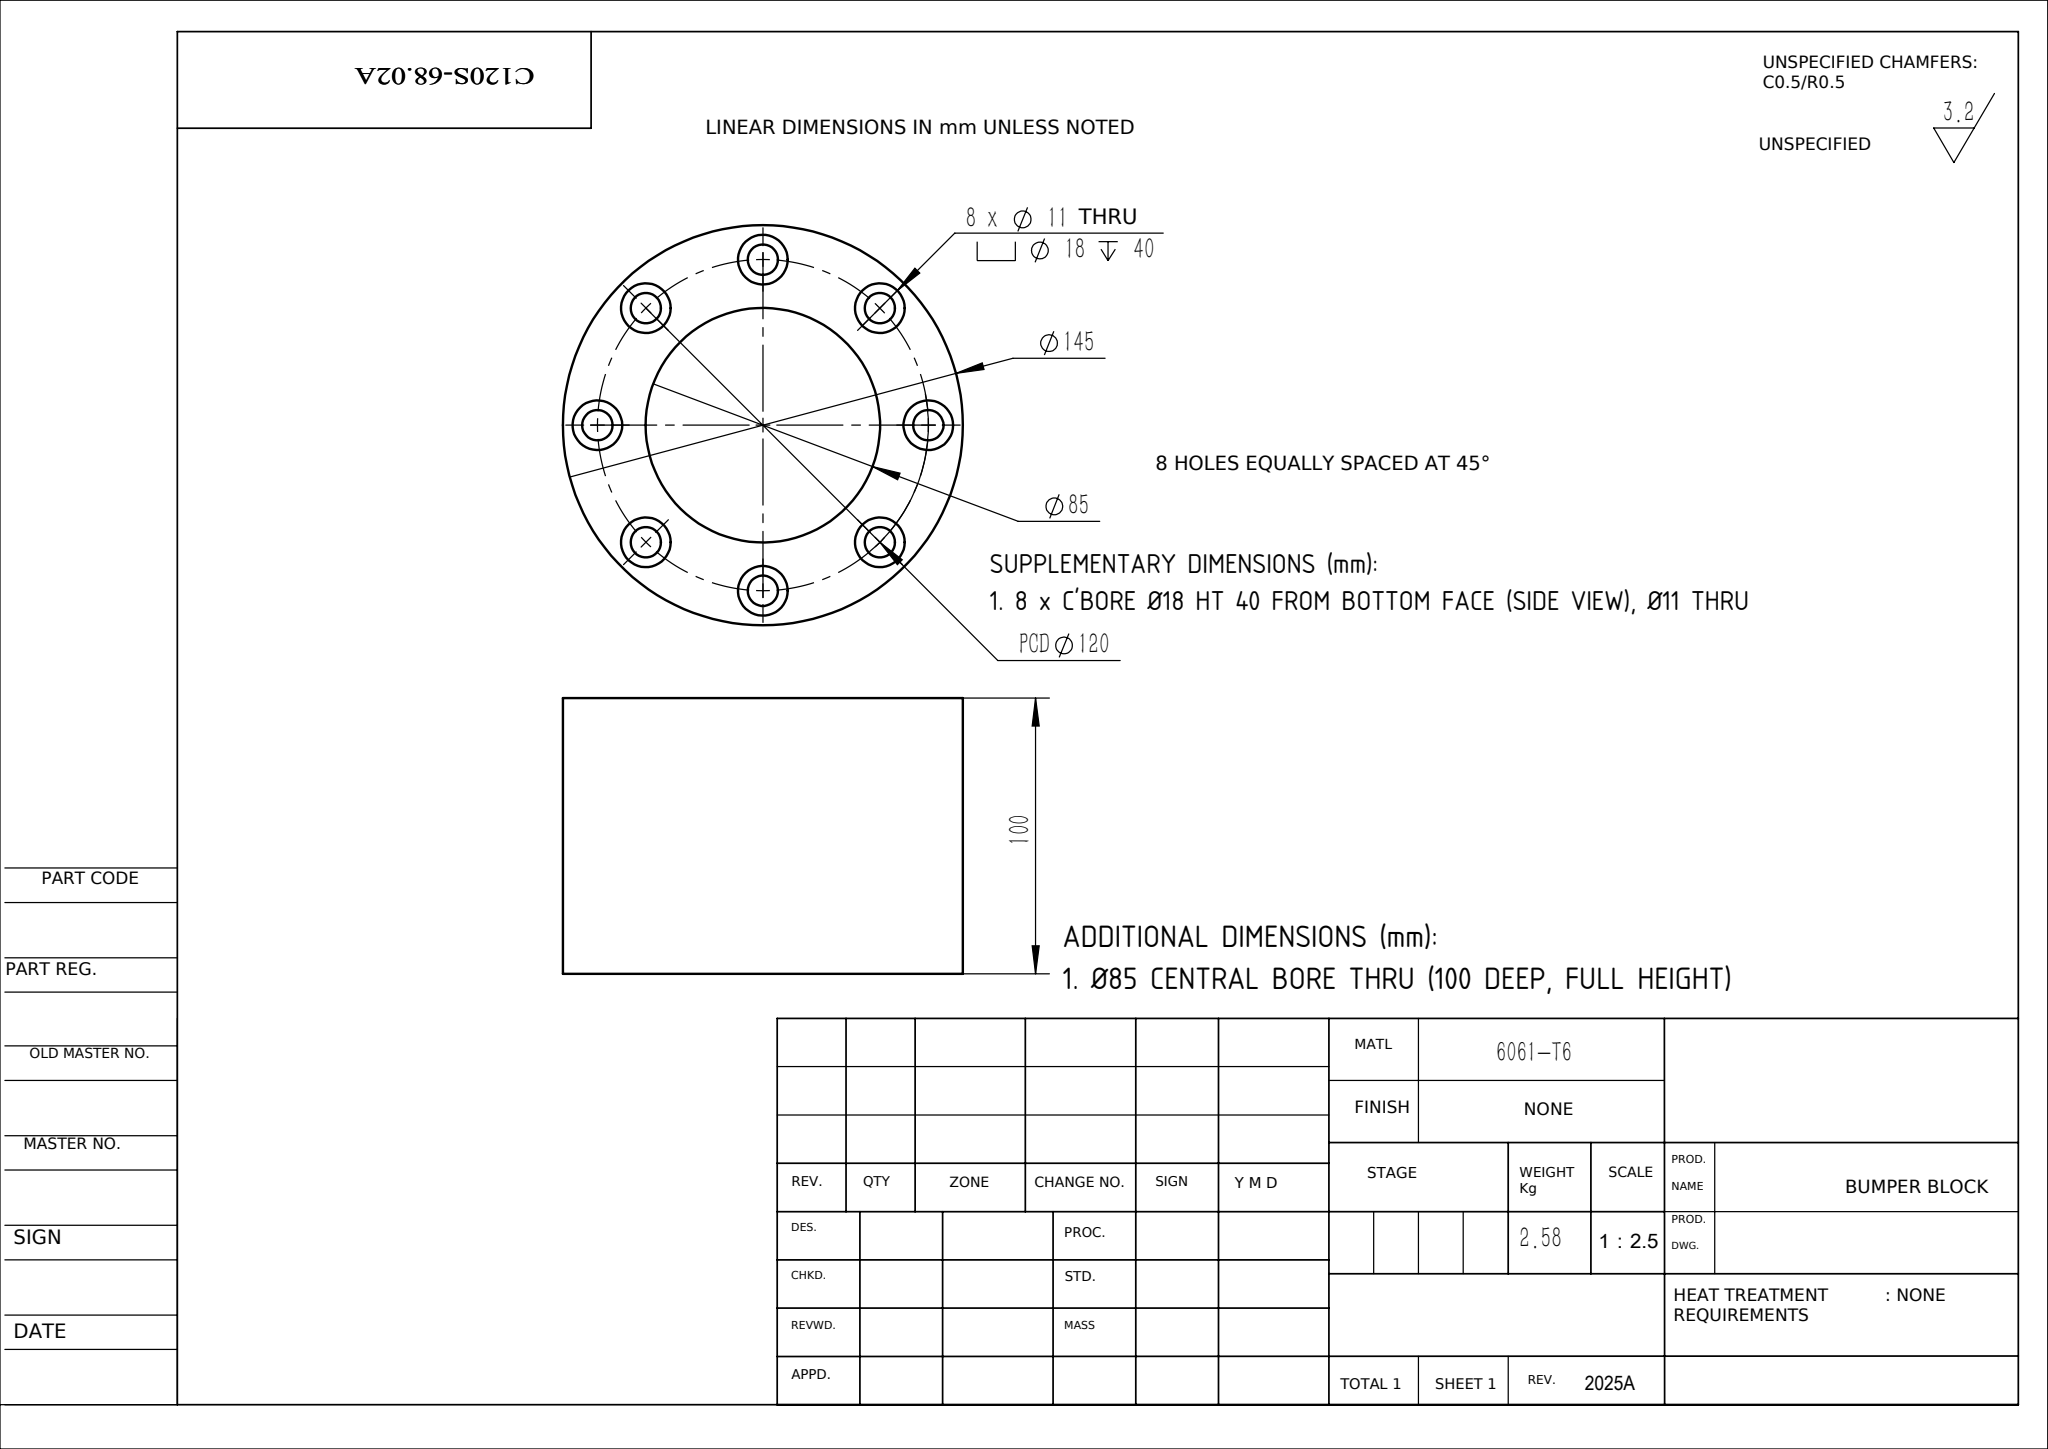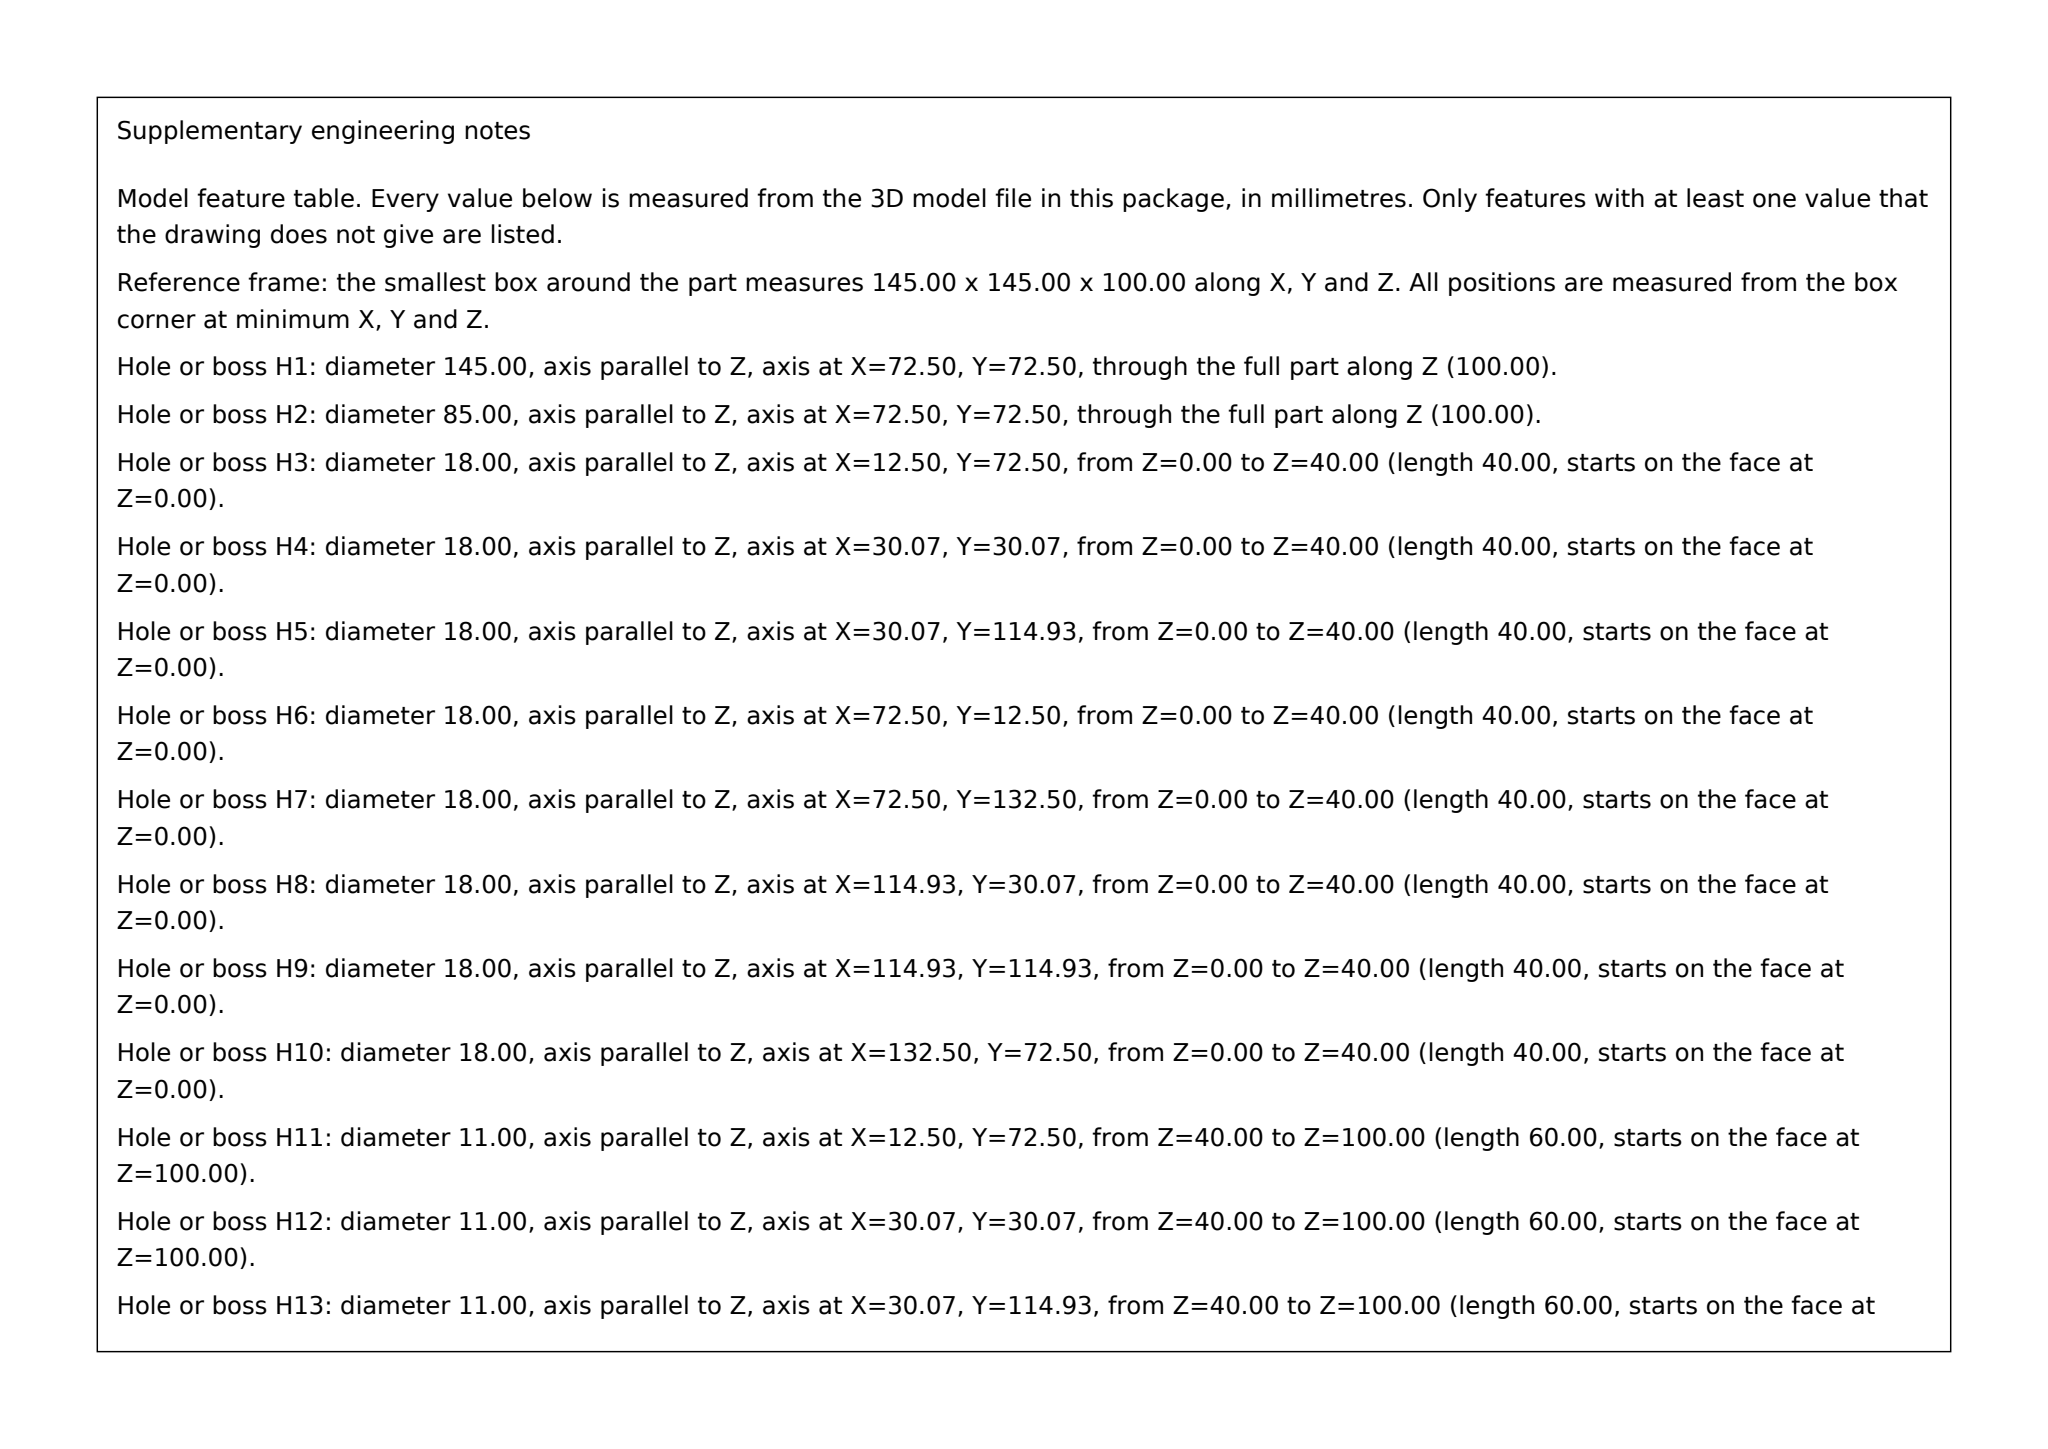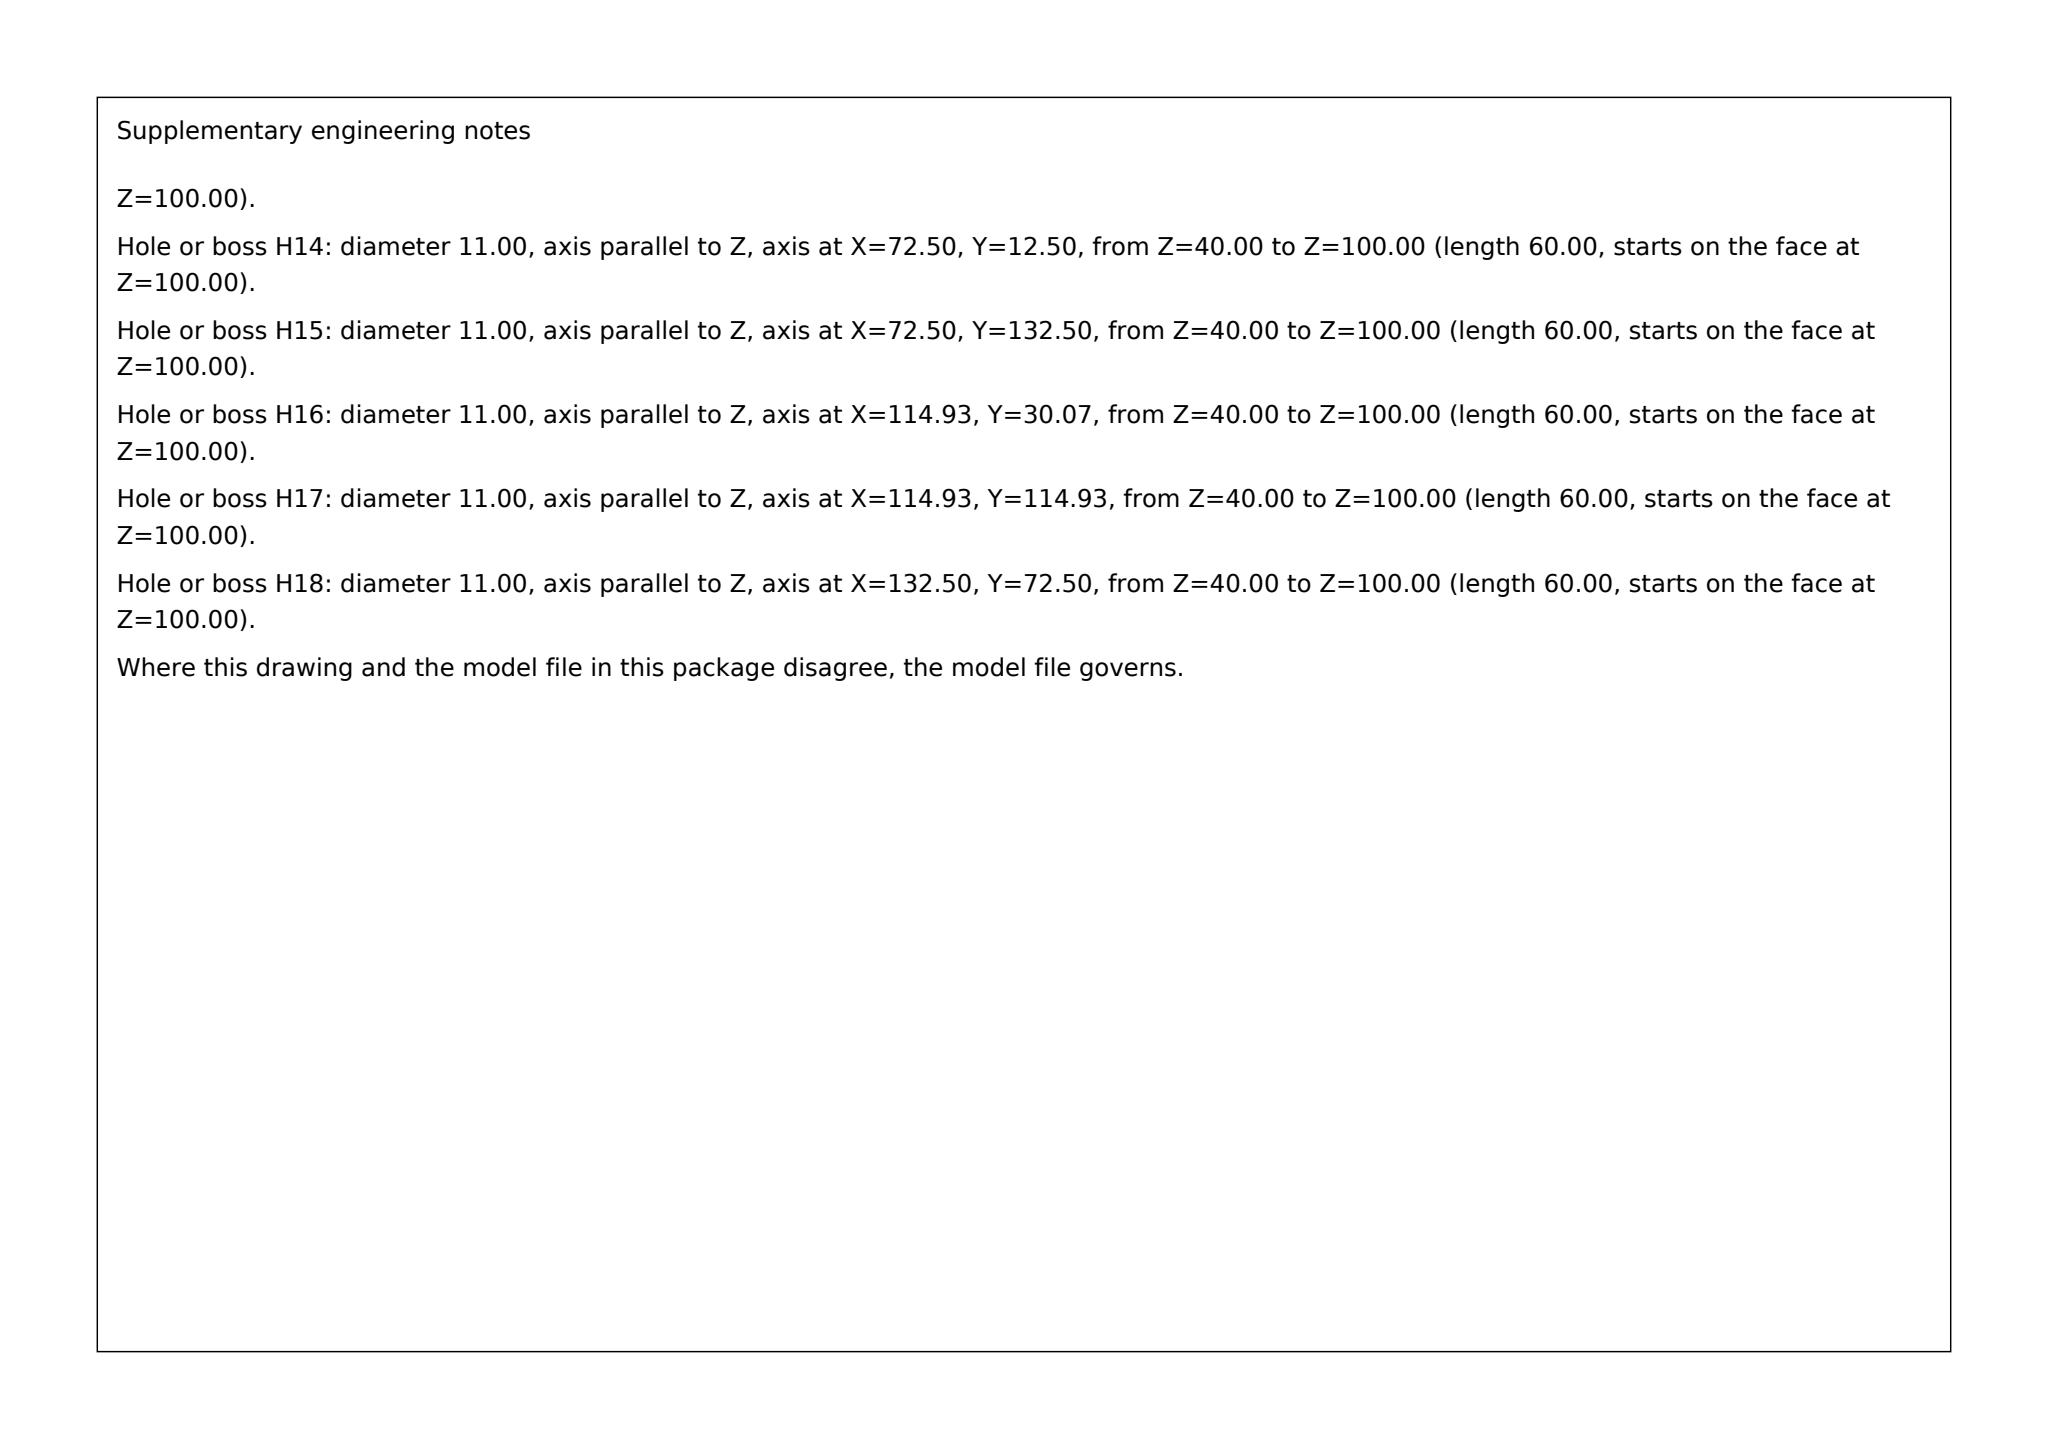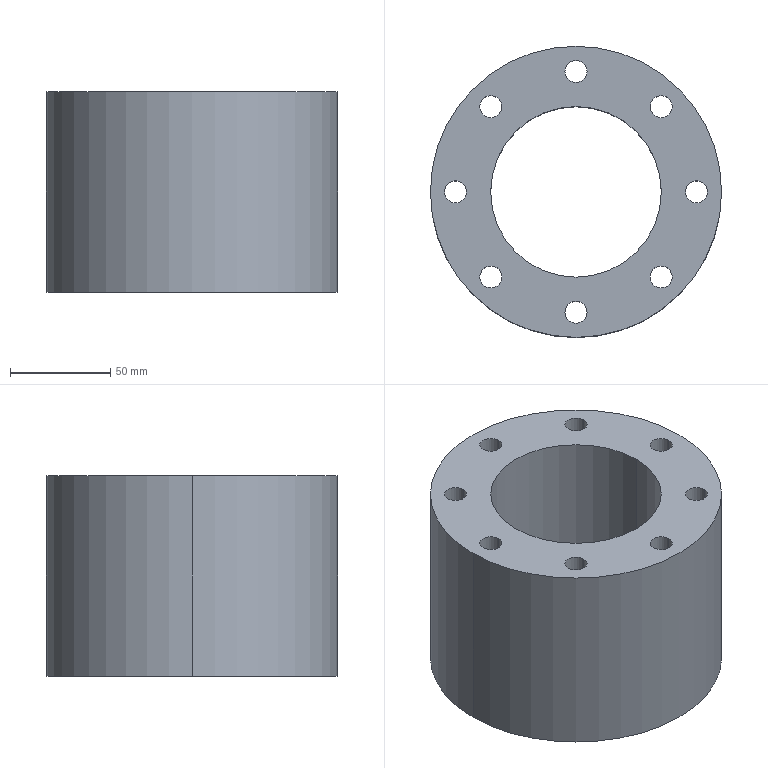Part | SolidWorks | mm | 1 solid | 46 faces | box 145 x 145 x 100 mm | volume 956803 mm3 | cylinder 36 | plane 10 | commonest cylinder face diameters 18 x16 11 x16 85 x2 145 x2
build123d program:
from build123d import *

# Parameters (mm, degrees)
SKETCH1_R                                         = 72.5
SKETCH1_R_2                                       = 42.5
BOSS_EXTRUDE1_DEPTH                               = 100
HOLE_SIZE_ACCORDING_TO_HEXAGON_SOCKET_D           = 11
HOLE_SIZE_ACCORDING_TO_HEXAGON_SOCKET_CBORE_D     = 18
HOLE_SIZE_ACCORDING_TO_HEXAGON_SOCKET_CBORE_DEPTH = 40
CIRPATTERN1_COUNT                                 = 8


with BuildPart() as part:
    # Sketch1 → Boss-Extrude1 (new body)
    with BuildSketch(Plane.XY):
        Circle(SKETCH1_R)
        Circle(SKETCH1_R_2, mode=Mode.SUBTRACT)
    extrude(amount=BOSS_EXTRUDE1_DEPTH)

    # Hole Size _ according to_ Hexagon Socket (through all)
    with Locations(Plane(origin=(0, 0, 0), x_dir=(-1, 0, 0), z_dir=(0, 0, -1))):
        with Locations((0, 60)):
            hole_size_according_to_hexagon_socket = CounterBoreHole(HOLE_SIZE_ACCORDING_TO_HEXAGON_SOCKET_D / 2, HOLE_SIZE_ACCORDING_TO_HEXAGON_SOCKET_CBORE_D / 2, HOLE_SIZE_ACCORDING_TO_HEXAGON_SOCKET_CBORE_DEPTH)

    # CirPattern1: Hole Size _ according to_ Hexagon Socket ×8 about axis
    cirpattern1_axis = Axis((0, 0, 0), (0, 0, 1))
    for i in range(1, CIRPATTERN1_COUNT):
        add(hole_size_according_to_hexagon_socket.rotate(cirpattern1_axis, i * 360 / CIRPATTERN1_COUNT), mode=Mode.SUBTRACT)


solid = part.part